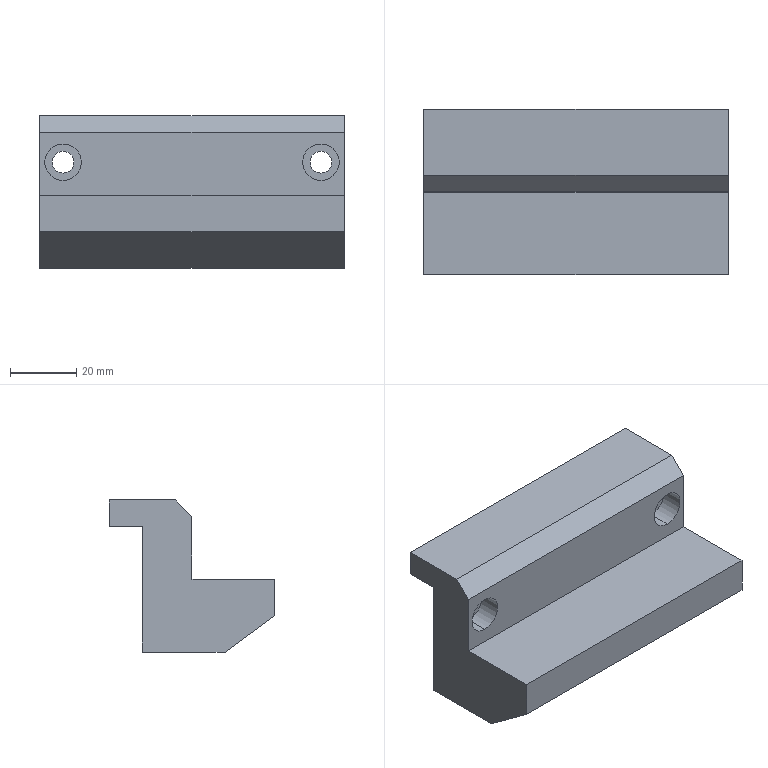Component | SolidWorks | RetractableStop-LongSide-1_AlignmentStop-0510-1 | 1 solid | 22 faces | box 92 x 50 x 46 mm | volume 110846 mm3 | plane 14 | cylinder 8 | commonest cylinder face diameters 11 x4 6.6 x4
build123d program:
from build123d import *

# Parameters (mm, degrees)
SKETCH1_W                                            = 92
SKETCH1_H                                            = 15
BOSS_EXTRUDE1_DEPTH                                  = 46
HOLE_SIZE_ACCORDING_TO_HEX_SOCKET_HEAD_C_D           = 6.6
HOLE_SIZE_ACCORDING_TO_HEX_SOCKET_HEAD_C_CBORE_D     = 11
HOLE_SIZE_ACCORDING_TO_HEX_SOCKET_HEAD_C_CBORE_DEPTH = 6.8
SKETCH11_W                                           = 92
SKETCH11_H                                           = 22
BOSS_EXTRUDE2_DEPTH                                  = 25
SKETCH12_W                                           = 92
SKETCH12_H                                           = 8
BOSS_EXTRUDE3_DEPTH                                  = 10
CUT_EXTRUDE1_DEPTH                                   = 106.854
CHAMFER1_SIZE                                        = 5


with BuildPart() as part:
    # Sketch1 → Boss-Extrude1 (new body)
    with BuildSketch(Plane.XY):
        with Locations((46, -7.5)):
            Rectangle(SKETCH1_W, SKETCH1_H)
    extrude(amount=BOSS_EXTRUDE1_DEPTH)

    # Hole Size according to Hex Socket Head C (through all)
    with Locations(Plane(origin=(0, 0, 0), x_dir=(1, 0, 0), z_dir=(0, 1, 0))):
        with Locations((7, -14), (85, -14)):
            CounterBoreHole(HOLE_SIZE_ACCORDING_TO_HEX_SOCKET_HEAD_C_D / 2, HOLE_SIZE_ACCORDING_TO_HEX_SOCKET_HEAD_C_CBORE_D / 2, HOLE_SIZE_ACCORDING_TO_HEX_SOCKET_HEAD_C_CBORE_DEPTH)

    # Sketch11 → Boss-Extrude2 (add)
    with BuildSketch(Plane(origin=(0, 0, 0), x_dir=(1, 0, 0), z_dir=(0, 1, 0))):
        with Locations((46, -35)):
            Rectangle(SKETCH11_W, SKETCH11_H)
    extrude(amount=BOSS_EXTRUDE2_DEPTH)

    # Sketch12 → Boss-Extrude3 (add)
    with BuildSketch(Plane.XZ.offset(15)):
        with Locations((46, 4)):
            Rectangle(SKETCH12_W, SKETCH12_H)
    extrude(amount=BOSS_EXTRUDE3_DEPTH)

    # Sketch13 → Cut-Extrude1 (cut, through all)
    with BuildSketch(Plane.ZY):
        Polygon((35, 25), (46, 10), (46, 25), align=None)
    extrude(amount=-CUT_EXTRUDE1_DEPTH, mode=Mode.SUBTRACT)

    # Chamfer1
    chamfer1_edges = [part.edges().sort_by_distance(p)[0] for p in [
        (46, 0, 0),
    ]]
    chamfer(chamfer1_edges, length=CHAMFER1_SIZE)


solid = part.part

# Placed as in the assembly
solid = solid.moved(Location((-1378.013, -21.764, 3640.5), (180, 0, 0)))
STEP:
#1=CARTESIAN_POINT('',(-53.977,-0.5891,142.992));
#2=VERTEX_POINT('',#1);
#3=CARTESIAN_POINT('',(-53.977,-0.5891,142.559));
#4=VERTEX_POINT('',#3);
#5=CARTESIAN_POINT('',(-53.977,-0.5891,142.776));
#6=DIRECTION('',(0.,-1.,0.));
#7=DIRECTION('',(0.,-0.,-1.));
#8=AXIS2_PLACEMENT_3D('',#5,#6,#7);
#9=CIRCLE('',#8,0.2165);
#10=EDGE_CURVE('',#2,#4,#9,.T.);
#11=ORIENTED_EDGE('',*,*,#10,.F.);
#12=CARTESIAN_POINT('',(-53.977,-0.8568,142.992));
#13=VERTEX_POINT('',#12);
#14=CARTESIAN_POINT('',(-53.977,-0.8568,142.992));
#15=DIRECTION('',(0.,-1.,0.));
#16=VECTOR('',#15,39.37);
#17=LINE('',#14,#16);
#18=EDGE_CURVE('',#2,#13,#17,.T.);
#19=ORIENTED_EDGE('',*,*,#18,.T.);
#20=CARTESIAN_POINT('',(-53.977,-0.8568,142.559));
#21=VERTEX_POINT('',#20);
#22=CARTESIAN_POINT('',(-53.977,-0.8568,142.776));
#23=DIRECTION('',(0.,-1.,0.));
#24=DIRECTION('',(0.,0.,-1.));
#25=AXIS2_PLACEMENT_3D('',#22,#23,#24);
#26=CIRCLE('',#25,0.2165);
#27=EDGE_CURVE('',#13,#21,#26,.T.);
#28=ORIENTED_EDGE('',*,*,#27,.T.);
#29=CARTESIAN_POINT('',(-53.977,-0.8568,142.559));
#30=DIRECTION('',(0.,-1.,0.));
#31=VECTOR('',#30,39.37);
#32=LINE('',#29,#31);
#33=EDGE_CURVE('',#4,#21,#32,.T.);
#34=ORIENTED_EDGE('',*,*,#33,.F.);
#35=EDGE_LOOP('',(#11,#19,#28,#34));
#36=FACE_OUTER_BOUND('',#35,.T.);
#37=CARTESIAN_POINT('',(-53.977,-0.8568,142.776));
#38=DIRECTION('',(0.,-1.,0.));
#39=DIRECTION('',(0.,0.,-1.));
#40=AXIS2_PLACEMENT_3D('',#37,#38,#39);
#41=CYLINDRICAL_SURFACE('',#40,0.2165);
#42=ADVANCED_FACE('',(#36),#41,.F.);
#43=CARTESIAN_POINT('',(-53.977,-0.2663,142.906));
#44=VERTEX_POINT('',#43);
#45=CARTESIAN_POINT('',(-53.977,-0.2663,142.646));
#46=VERTEX_POINT('',#45);
#47=CARTESIAN_POINT('',(-53.977,-0.2663,142.776));
#48=DIRECTION('',(0.,-1.,0.));
#49=DIRECTION('',(0.,-0.,-1.));
#50=AXIS2_PLACEMENT_3D('',#47,#48,#49);
#51=CIRCLE('',#50,0.1299);
#52=EDGE_CURVE('',#44,#46,#51,.T.);
#53=ORIENTED_EDGE('',*,*,#52,.F.);
#54=CARTESIAN_POINT('',(-53.977,-0.5891,142.906));
#55=VERTEX_POINT('',#54);
#56=CARTESIAN_POINT('',(-53.977,-0.8568,142.906));
#57=DIRECTION('',(0.,-1.,0.));
#58=VECTOR('',#57,39.37);
#59=LINE('',#56,#58);
#60=EDGE_CURVE('',#44,#55,#59,.T.);
#61=ORIENTED_EDGE('',*,*,#60,.T.);
#62=CARTESIAN_POINT('',(-53.977,-0.5891,142.646));
#63=VERTEX_POINT('',#62);
#64=CARTESIAN_POINT('',(-53.977,-0.5891,142.776));
#65=DIRECTION('',(0.,-1.,0.));
#66=DIRECTION('',(0.,-0.,-1.));
#67=AXIS2_PLACEMENT_3D('',#64,#65,#66);
#68=CIRCLE('',#67,0.1299);
#69=EDGE_CURVE('',#55,#63,#68,.T.);
#70=ORIENTED_EDGE('',*,*,#69,.T.);
#71=CARTESIAN_POINT('',(-53.977,-0.8568,142.646));
#72=DIRECTION('',(0.,-1.,0.));
#73=VECTOR('',#72,39.37);
#74=LINE('',#71,#73);
#75=EDGE_CURVE('',#46,#63,#74,.T.);
#76=ORIENTED_EDGE('',*,*,#75,.F.);
#77=EDGE_LOOP('',(#53,#61,#70,#76));
#78=FACE_OUTER_BOUND('',#77,.T.);
#79=CARTESIAN_POINT('',(-53.977,-0.8568,142.776));
#80=DIRECTION('',(0.,-1.,0.));
#81=DIRECTION('',(0.,0.,-1.));
#82=AXIS2_PLACEMENT_3D('',#79,#80,#81);
#83=CYLINDRICAL_SURFACE('',#82,0.1299);
#84=ADVANCED_FACE('',(#78),#83,.F.);
#85=CARTESIAN_POINT('',(-50.906,-0.5891,142.992));
#86=VERTEX_POINT('',#85);
#87=CARTESIAN_POINT('',(-50.906,-0.5891,142.559));
#88=VERTEX_POINT('',#87);
#89=CARTESIAN_POINT('',(-50.906,-0.5891,142.776));
#90=DIRECTION('',(0.,-1.,0.));
#91=DIRECTION('',(0.,-0.,-1.));
#92=AXIS2_PLACEMENT_3D('',#89,#90,#91);
#93=CIRCLE('',#92,0.2165);
#94=EDGE_CURVE('',#86,#88,#93,.T.);
#95=ORIENTED_EDGE('',*,*,#94,.F.);
#96=CARTESIAN_POINT('',(-50.906,-0.8568,142.992));
#97=VERTEX_POINT('',#96);
#98=CARTESIAN_POINT('',(-50.906,-0.8568,142.992));
#99=DIRECTION('',(0.,-1.,0.));
#100=VECTOR('',#99,39.37);
#101=LINE('',#98,#100);
#102=EDGE_CURVE('',#86,#97,#101,.T.);
#103=ORIENTED_EDGE('',*,*,#102,.T.);
#104=CARTESIAN_POINT('',(-50.906,-0.8568,142.559));
#105=VERTEX_POINT('',#104);
#106=CARTESIAN_POINT('',(-50.906,-0.8568,142.776));
#107=DIRECTION('',(0.,-1.,0.));
#108=DIRECTION('',(0.,0.,-1.));
#109=AXIS2_PLACEMENT_3D('',#106,#107,#108);
#110=CIRCLE('',#109,0.2165);
#111=EDGE_CURVE('',#97,#105,#110,.T.);
#112=ORIENTED_EDGE('',*,*,#111,.T.);
#113=CARTESIAN_POINT('',(-50.906,-0.8568,142.559));
#114=DIRECTION('',(0.,-1.,0.));
#115=VECTOR('',#114,39.37);
#116=LINE('',#113,#115);
#117=EDGE_CURVE('',#88,#105,#116,.T.);
#118=ORIENTED_EDGE('',*,*,#117,.F.);
#119=EDGE_LOOP('',(#95,#103,#112,#118));
#120=FACE_OUTER_BOUND('',#119,.T.);
#121=CARTESIAN_POINT('',(-50.906,-0.8568,142.776));
#122=DIRECTION('',(0.,-1.,0.));
#123=DIRECTION('',(0.,0.,-1.));
#124=AXIS2_PLACEMENT_3D('',#121,#122,#123);
#125=CYLINDRICAL_SURFACE('',#124,0.2165);
#126=ADVANCED_FACE('',(#120),#125,.F.);
#127=CARTESIAN_POINT('',(-50.906,-0.2663,142.906));
#128=VERTEX_POINT('',#127);
#129=CARTESIAN_POINT('',(-50.906,-0.2663,142.646));
#130=VERTEX_POINT('',#129);
#131=CARTESIAN_POINT('',(-50.906,-0.2663,142.776));
#132=DIRECTION('',(0.,-1.,0.));
#133=DIRECTION('',(0.,-0.,-1.));
#134=AXIS2_PLACEMENT_3D('',#131,#132,#133);
#135=CIRCLE('',#134,0.1299);
#136=EDGE_CURVE('',#128,#130,#135,.T.);
#137=ORIENTED_EDGE('',*,*,#136,.F.);
#138=CARTESIAN_POINT('',(-50.906,-0.5891,142.906));
#139=VERTEX_POINT('',#138);
#140=CARTESIAN_POINT('',(-50.906,-0.8568,142.906));
#141=DIRECTION('',(0.,-1.,0.));
#142=VECTOR('',#141,39.37);
#143=LINE('',#140,#142);
#144=EDGE_CURVE('',#128,#139,#143,.T.);
#145=ORIENTED_EDGE('',*,*,#144,.T.);
#146=CARTESIAN_POINT('',(-50.906,-0.5891,142.646));
#147=VERTEX_POINT('',#146);
#148=CARTESIAN_POINT('',(-50.906,-0.5891,142.776));
#149=DIRECTION('',(0.,-1.,0.));
#150=DIRECTION('',(0.,-0.,-1.));
#151=AXIS2_PLACEMENT_3D('',#148,#149,#150);
#152=CIRCLE('',#151,0.1299);
#153=EDGE_CURVE('',#139,#147,#152,.T.);
#154=ORIENTED_EDGE('',*,*,#153,.T.);
#155=CARTESIAN_POINT('',(-50.906,-0.8568,142.646));
#156=DIRECTION('',(0.,-1.,0.));
#157=VECTOR('',#156,39.37);
#158=LINE('',#155,#157);
#159=EDGE_CURVE('',#130,#147,#158,.T.);
#160=ORIENTED_EDGE('',*,*,#159,.F.);
#161=EDGE_LOOP('',(#137,#145,#154,#160));
#162=FACE_OUTER_BOUND('',#161,.T.);
#163=CARTESIAN_POINT('',(-50.906,-0.8568,142.776));
#164=DIRECTION('',(0.,-1.,0.));
#165=DIRECTION('',(0.,0.,-1.));
#166=AXIS2_PLACEMENT_3D('',#163,#164,#165);
#167=CYLINDRICAL_SURFACE('',#166,0.1299);
#168=ADVANCED_FACE('',(#162),#167,.F.);
#169=CARTESIAN_POINT('',(-50.906,-0.2663,142.776));
#170=DIRECTION('',(0.,-1.,0.));
#171=DIRECTION('',(0.,-0.,-1.));
#172=AXIS2_PLACEMENT_3D('',#169,#170,#171);
#173=CIRCLE('',#172,0.1299);
#174=EDGE_CURVE('',#130,#128,#173,.T.);
#175=ORIENTED_EDGE('',*,*,#174,.T.);
#176=ORIENTED_EDGE('',*,*,#136,.T.);
#177=EDGE_LOOP('',(#175,#176));
#178=FACE_BOUND('',#177,.T.);
#179=CARTESIAN_POINT('',(-53.977,-0.2663,142.776));
#180=DIRECTION('',(0.,-1.,0.));
#181=DIRECTION('',(0.,-0.,-1.));
#182=AXIS2_PLACEMENT_3D('',#179,#180,#181);
#183=CIRCLE('',#182,0.1299);
#184=EDGE_CURVE('',#46,#44,#183,.T.);
#185=ORIENTED_EDGE('',*,*,#184,.T.);
#186=ORIENTED_EDGE('',*,*,#52,.T.);
#187=EDGE_LOOP('',(#185,#186));
#188=FACE_BOUND('',#187,.T.);
#189=CARTESIAN_POINT('',(-50.63,-0.2663,143.012));
#190=VERTEX_POINT('',#189);
#191=CARTESIAN_POINT('',(-54.252,-0.2663,143.012));
#192=VERTEX_POINT('',#191);
#193=CARTESIAN_POINT('',(-54.252,-0.2663,143.012));
#194=DIRECTION('',(-1.,-0.,0.));
#195=VECTOR('',#194,39.37);
#196=LINE('',#193,#195);
#197=EDGE_CURVE('',#190,#192,#196,.T.);
#198=ORIENTED_EDGE('',*,*,#197,.F.);
#199=CARTESIAN_POINT('',(-50.63,-0.2663,141.516));
#200=VERTEX_POINT('',#199);
#201=CARTESIAN_POINT('',(-50.63,-0.2663,141.516));
#202=DIRECTION('',(0.,0.,1.));
#203=VECTOR('',#202,39.37);
#204=LINE('',#201,#203);
#205=EDGE_CURVE('',#200,#190,#204,.T.);
#206=ORIENTED_EDGE('',*,*,#205,.F.);
#207=CARTESIAN_POINT('',(-54.252,-0.2663,141.516));
#208=VERTEX_POINT('',#207);
#209=CARTESIAN_POINT('',(-54.252,-0.2663,141.516));
#210=DIRECTION('',(1.,0.,-0.));
#211=VECTOR('',#210,39.37);
#212=LINE('',#209,#211);
#213=EDGE_CURVE('',#208,#200,#212,.T.);
#214=ORIENTED_EDGE('',*,*,#213,.F.);
#215=CARTESIAN_POINT('',(-54.252,-0.2663,141.516));
#216=DIRECTION('',(0.,0.,1.));
#217=VECTOR('',#216,39.37);
#218=LINE('',#215,#217);
#219=EDGE_CURVE('',#208,#192,#218,.T.);
#220=ORIENTED_EDGE('',*,*,#219,.T.);
#221=EDGE_LOOP('',(#198,#206,#214,#220));
#222=FACE_OUTER_BOUND('',#221,.T.);
#223=CARTESIAN_POINT('',(-54.252,-0.2663,141.516));
#224=DIRECTION('',(0.,-1.,0.));
#225=DIRECTION('',(-1.,-0.,0.));
#226=AXIS2_PLACEMENT_3D('',#223,#224,#225);
#227=PLANE('',#226);
#228=ADVANCED_FACE('',(#178,#188,#222),#227,.F.);
#229=CARTESIAN_POINT('',(-50.906,-0.8568,142.776));
#230=DIRECTION('',(0.,-1.,0.));
#231=DIRECTION('',(0.,0.,-1.));
#232=AXIS2_PLACEMENT_3D('',#229,#230,#231);
#233=CIRCLE('',#232,0.2165);
#234=EDGE_CURVE('',#105,#97,#233,.T.);
#235=ORIENTED_EDGE('',*,*,#234,.F.);
#236=ORIENTED_EDGE('',*,*,#111,.F.);
#237=EDGE_LOOP('',(#235,#236));
#238=FACE_BOUND('',#237,.T.);
#239=CARTESIAN_POINT('',(-53.977,-0.8568,142.776));
#240=DIRECTION('',(0.,-1.,0.));
#241=DIRECTION('',(0.,0.,-1.));
#242=AXIS2_PLACEMENT_3D('',#239,#240,#241);
#243=CIRCLE('',#242,0.2165);
#244=EDGE_CURVE('',#21,#13,#243,.T.);
#245=ORIENTED_EDGE('',*,*,#244,.F.);
#246=ORIENTED_EDGE('',*,*,#27,.F.);
#247=EDGE_LOOP('',(#245,#246));
#248=FACE_BOUND('',#247,.T.);
#249=CARTESIAN_POINT('',(-50.63,-0.8568,142.382));
#250=VERTEX_POINT('',#249);
#251=CARTESIAN_POINT('',(-50.63,-0.8568,143.13));
#252=VERTEX_POINT('',#251);
#253=CARTESIAN_POINT('',(-50.63,-0.8568,141.516));
#254=DIRECTION('',(0.,0.,1.));
#255=VECTOR('',#254,39.37);
#256=LINE('',#253,#255);
#257=EDGE_CURVE('',#250,#252,#256,.T.);
#258=ORIENTED_EDGE('',*,*,#257,.T.);
#259=CARTESIAN_POINT('',(-54.252,-0.8568,143.13));
#260=VERTEX_POINT('',#259);
#261=CARTESIAN_POINT('',(-50.63,-0.8568,143.13));
#262=DIRECTION('',(-1.,0.,0.));
#263=VECTOR('',#262,39.37);
#264=LINE('',#261,#263);
#265=EDGE_CURVE('',#252,#260,#264,.T.);
#266=ORIENTED_EDGE('',*,*,#265,.T.);
#267=CARTESIAN_POINT('',(-54.252,-0.8568,142.382));
#268=VERTEX_POINT('',#267);
#269=CARTESIAN_POINT('',(-54.252,-0.8568,141.516));
#270=DIRECTION('',(0.,0.,1.));
#271=VECTOR('',#270,39.37);
#272=LINE('',#269,#271);
#273=EDGE_CURVE('',#268,#260,#272,.T.);
#274=ORIENTED_EDGE('',*,*,#273,.F.);
#275=CARTESIAN_POINT('',(-54.252,-0.8568,142.382));
#276=DIRECTION('',(-1.,0.,0.));
#277=VECTOR('',#276,39.37);
#278=LINE('',#275,#277);
#279=EDGE_CURVE('',#250,#268,#278,.T.);
#280=ORIENTED_EDGE('',*,*,#279,.F.);
#281=EDGE_LOOP('',(#258,#266,#274,#280));
#282=FACE_OUTER_BOUND('',#281,.T.);
#283=CARTESIAN_POINT('',(-50.63,-0.8568,141.516));
#284=DIRECTION('',(0.,1.,-0.));
#285=DIRECTION('',(1.,-0.,-0.));
#286=AXIS2_PLACEMENT_3D('',#283,#284,#285);
#287=PLANE('',#286);
#288=ADVANCED_FACE('',(#238,#248,#282),#287,.F.);
#289=CARTESIAN_POINT('',(-50.63,0.1274,143.327));
#290=VERTEX_POINT('',#289);
#291=CARTESIAN_POINT('',(-50.63,-0.66,143.327));
#292=VERTEX_POINT('',#291);
#293=CARTESIAN_POINT('',(-50.63,-0.2663,143.327));
#294=DIRECTION('',(0.,-1.,0.));
#295=VECTOR('',#294,39.37);
#296=LINE('',#293,#295);
#297=EDGE_CURVE('',#290,#292,#296,.T.);
#298=ORIENTED_EDGE('',*,*,#297,.T.);
#299=CARTESIAN_POINT('',(-50.63,-0.8568,143.13));
#300=DIRECTION('',(-0.,-0.7071,-0.7071));
#301=VECTOR('',#300,39.37);
#302=LINE('',#299,#301);
#303=EDGE_CURVE('',#292,#252,#302,.T.);
#304=ORIENTED_EDGE('',*,*,#303,.T.);
#305=ORIENTED_EDGE('',*,*,#257,.F.);
#306=CARTESIAN_POINT('',(-50.63,-1.841,142.382));
#307=VERTEX_POINT('',#306);
#308=CARTESIAN_POINT('',(-50.63,-1.841,142.382));
#309=DIRECTION('',(0.,1.,-0.));
#310=VECTOR('',#309,39.37);
#311=LINE('',#308,#310);
#312=EDGE_CURVE('',#307,#250,#311,.T.);
#313=ORIENTED_EDGE('',*,*,#312,.F.);
#314=CARTESIAN_POINT('',(-50.63,-1.841,141.949));
#315=VERTEX_POINT('',#314);
#316=CARTESIAN_POINT('',(-50.63,-1.841,141.516));
#317=DIRECTION('',(0.,0.,1.));
#318=VECTOR('',#317,39.37);
#319=LINE('',#316,#318);
#320=EDGE_CURVE('',#315,#307,#319,.T.);
#321=ORIENTED_EDGE('',*,*,#320,.F.);
#322=CARTESIAN_POINT('',(-50.63,-1.251,141.516));
#323=VERTEX_POINT('',#322);
#324=CARTESIAN_POINT('',(-50.63,-0.6105,141.046));
#325=DIRECTION('',(-0.,0.8064,-0.5914));
#326=VECTOR('',#325,39.37);
#327=LINE('',#324,#326);
#328=EDGE_CURVE('',#315,#323,#327,.T.);
#329=ORIENTED_EDGE('',*,*,#328,.T.);
#330=CARTESIAN_POINT('',(-50.63,-0.2663,141.516));
#331=DIRECTION('',(0.,-1.,0.));
#332=VECTOR('',#331,39.37);
#333=LINE('',#330,#332);
#334=EDGE_CURVE('',#200,#323,#333,.T.);
#335=ORIENTED_EDGE('',*,*,#334,.F.);
#336=ORIENTED_EDGE('',*,*,#205,.T.);
#337=CARTESIAN_POINT('',(-50.63,0.1274,143.012));
#338=VERTEX_POINT('',#337);
#339=CARTESIAN_POINT('',(-50.63,0.1274,143.012));
#340=DIRECTION('',(0.,-1.,0.));
#341=VECTOR('',#340,39.37);
#342=LINE('',#339,#341);
#343=EDGE_CURVE('',#338,#190,#342,.T.);
#344=ORIENTED_EDGE('',*,*,#343,.F.);
#345=CARTESIAN_POINT('',(-50.63,0.1274,143.327));
#346=DIRECTION('',(-0.,-0.,-1.));
#347=VECTOR('',#346,39.37);
#348=LINE('',#345,#347);
#349=EDGE_CURVE('',#290,#338,#348,.T.);
#350=ORIENTED_EDGE('',*,*,#349,.F.);
#351=EDGE_LOOP('',(#298,#304,#305,#313,#321,#329,#335,#336,#344,#350));
#352=FACE_OUTER_BOUND('',#351,.T.);
#353=CARTESIAN_POINT('',(-50.63,-0.2663,141.516));
#354=DIRECTION('',(-1.,-0.,0.));
#355=DIRECTION('',(-0.,-0.,-1.));
#356=AXIS2_PLACEMENT_3D('',#353,#354,#355);
#357=PLANE('',#356);
#358=ADVANCED_FACE('',(#352),#357,.F.);
#359=ORIENTED_EDGE('',*,*,#273,.T.);
#360=CARTESIAN_POINT('',(-54.252,-0.66,143.327));
#361=VERTEX_POINT('',#360);
#362=CARTESIAN_POINT('',(-54.252,-0.8568,143.13));
#363=DIRECTION('',(0.,0.7071,0.7071));
#364=VECTOR('',#363,39.37);
#365=LINE('',#362,#364);
#366=EDGE_CURVE('',#260,#361,#365,.T.);
#367=ORIENTED_EDGE('',*,*,#366,.T.);
#368=CARTESIAN_POINT('',(-54.252,0.1274,143.327));
#369=VERTEX_POINT('',#368);
#370=CARTESIAN_POINT('',(-54.252,-0.8568,143.327));
#371=DIRECTION('',(-0.,1.,-0.));
#372=VECTOR('',#371,39.37);
#373=LINE('',#370,#372);
#374=EDGE_CURVE('',#361,#369,#373,.T.);
#375=ORIENTED_EDGE('',*,*,#374,.T.);
#376=CARTESIAN_POINT('',(-54.252,0.1274,143.012));
#377=VERTEX_POINT('',#376);
#378=CARTESIAN_POINT('',(-54.252,0.1274,143.327));
#379=DIRECTION('',(0.,0.,1.));
#380=VECTOR('',#379,39.37);
#381=LINE('',#378,#380);
#382=EDGE_CURVE('',#377,#369,#381,.T.);
#383=ORIENTED_EDGE('',*,*,#382,.F.);
#384=CARTESIAN_POINT('',(-54.252,0.1274,143.012));
#385=DIRECTION('',(0.,-1.,0.));
#386=VECTOR('',#385,39.37);
#387=LINE('',#384,#386);
#388=EDGE_CURVE('',#377,#192,#387,.T.);
#389=ORIENTED_EDGE('',*,*,#388,.T.);
#390=ORIENTED_EDGE('',*,*,#219,.F.);
#391=CARTESIAN_POINT('',(-54.252,-1.251,141.516));
#392=VERTEX_POINT('',#391);
#393=CARTESIAN_POINT('',(-54.252,-0.8568,141.516));
#394=DIRECTION('',(-0.,1.,-0.));
#395=VECTOR('',#394,39.37);
#396=LINE('',#393,#395);
#397=EDGE_CURVE('',#392,#208,#396,.T.);
#398=ORIENTED_EDGE('',*,*,#397,.F.);
#399=CARTESIAN_POINT('',(-54.252,-1.841,141.949));
#400=VERTEX_POINT('',#399);
#401=CARTESIAN_POINT('',(-54.252,-1.841,141.949));
#402=DIRECTION('',(-0.,0.8064,-0.5914));
#403=VECTOR('',#402,39.37);
#404=LINE('',#401,#403);
#405=EDGE_CURVE('',#400,#392,#404,.T.);
#406=ORIENTED_EDGE('',*,*,#405,.F.);
#407=CARTESIAN_POINT('',(-54.252,-1.841,142.382));
#408=VERTEX_POINT('',#407);
#409=CARTESIAN_POINT('',(-54.252,-1.841,141.516));
#410=DIRECTION('',(-0.,-0.,-1.));
#411=VECTOR('',#410,39.37);
#412=LINE('',#409,#411);
#413=EDGE_CURVE('',#408,#400,#412,.T.);
#414=ORIENTED_EDGE('',*,*,#413,.F.);
#415=CARTESIAN_POINT('',(-54.252,-1.841,142.382));
#416=DIRECTION('',(0.,1.,-0.));
#417=VECTOR('',#416,39.37);
#418=LINE('',#415,#417);
#419=EDGE_CURVE('',#408,#268,#418,.T.);
#420=ORIENTED_EDGE('',*,*,#419,.T.);
#421=EDGE_LOOP('',(#359,#367,#375,#383,#389,#390,#398,#406,#414,#420));
#422=FACE_OUTER_BOUND('',#421,.T.);
#423=CARTESIAN_POINT('',(-54.252,-0.8568,141.516));
#424=DIRECTION('',(1.,0.,-0.));
#425=DIRECTION('',(0.,0.,1.));
#426=AXIS2_PLACEMENT_3D('',#423,#424,#425);
#427=PLANE('',#426);
#428=ADVANCED_FACE('',(#422),#427,.F.);
#429=CARTESIAN_POINT('',(-50.63,-1.251,141.516));
#430=DIRECTION('',(-1.,-0.,0.));
#431=VECTOR('',#430,39.37);
#432=LINE('',#429,#431);
#433=EDGE_CURVE('',#323,#392,#432,.T.);
#434=ORIENTED_EDGE('',*,*,#433,.T.);
#435=ORIENTED_EDGE('',*,*,#397,.T.);
#436=ORIENTED_EDGE('',*,*,#213,.T.);
#437=ORIENTED_EDGE('',*,*,#334,.T.);
#438=EDGE_LOOP('',(#434,#435,#436,#437));
#439=FACE_OUTER_BOUND('',#438,.T.);
#440=CARTESIAN_POINT('',(-54.252,-0.8568,141.516));
#441=DIRECTION('',(-0.,-0.,-1.));
#442=DIRECTION('',(1.,0.,-0.));
#443=AXIS2_PLACEMENT_3D('',#440,#441,#442);
#444=PLANE('',#443);
#445=ADVANCED_FACE('',(#439),#444,.T.);
#446=ORIENTED_EDGE('',*,*,#374,.F.);
#447=CARTESIAN_POINT('',(-54.252,-0.66,143.327));
#448=DIRECTION('',(1.,-0.,-0.));
#449=VECTOR('',#448,39.37);
#450=LINE('',#447,#449);
#451=EDGE_CURVE('',#361,#292,#450,.T.);
#452=ORIENTED_EDGE('',*,*,#451,.T.);
#453=ORIENTED_EDGE('',*,*,#297,.F.);
#454=CARTESIAN_POINT('',(-54.252,0.1274,143.327));
#455=DIRECTION('',(1.,0.,-0.));
#456=VECTOR('',#455,39.37);
#457=LINE('',#454,#456);
#458=EDGE_CURVE('',#369,#290,#457,.T.);
#459=ORIENTED_EDGE('',*,*,#458,.F.);
#460=EDGE_LOOP('',(#446,#452,#453,#459));
#461=FACE_OUTER_BOUND('',#460,.T.);
#462=CARTESIAN_POINT('',(-54.252,-0.8568,143.327));
#463=DIRECTION('',(-0.,-0.,-1.));
#464=DIRECTION('',(1.,0.,-0.));
#465=AXIS2_PLACEMENT_3D('',#462,#463,#464);
#466=PLANE('',#465);
#467=ADVANCED_FACE('',(#461),#466,.F.);
#468=ORIENTED_EDGE('',*,*,#144,.F.);
#469=ORIENTED_EDGE('',*,*,#174,.F.);
#470=ORIENTED_EDGE('',*,*,#159,.T.);
#471=CARTESIAN_POINT('',(-50.906,-0.5891,142.776));
#472=DIRECTION('',(0.,-1.,0.));
#473=DIRECTION('',(0.,-0.,-1.));
#474=AXIS2_PLACEMENT_3D('',#471,#472,#473);
#475=CIRCLE('',#474,0.1299);
#476=EDGE_CURVE('',#147,#139,#475,.T.);
#477=ORIENTED_EDGE('',*,*,#476,.T.);
#478=EDGE_LOOP('',(#468,#469,#470,#477));
#479=FACE_OUTER_BOUND('',#478,.T.);
#480=CARTESIAN_POINT('',(-50.906,-0.8568,142.776));
#481=DIRECTION('',(0.,-1.,0.));
#482=DIRECTION('',(0.,0.,-1.));
#483=AXIS2_PLACEMENT_3D('',#480,#481,#482);
#484=CYLINDRICAL_SURFACE('',#483,0.1299);
#485=ADVANCED_FACE('',(#479),#484,.F.);
#486=ORIENTED_EDGE('',*,*,#476,.F.);
#487=ORIENTED_EDGE('',*,*,#153,.F.);
#488=EDGE_LOOP('',(#486,#487));
#489=FACE_BOUND('',#488,.T.);
#490=CARTESIAN_POINT('',(-50.906,-0.5891,142.776));
#491=DIRECTION('',(0.,-1.,0.));
#492=DIRECTION('',(0.,-0.,-1.));
#493=AXIS2_PLACEMENT_3D('',#490,#491,#492);
#494=CIRCLE('',#493,0.2165);
#495=EDGE_CURVE('',#88,#86,#494,.T.);
#496=ORIENTED_EDGE('',*,*,#495,.T.);
#497=ORIENTED_EDGE('',*,*,#94,.T.);
#498=EDGE_LOOP('',(#496,#497));
#499=FACE_OUTER_BOUND('',#498,.T.);
#500=CARTESIAN_POINT('',(-50.776,-0.5891,142.776));
#501=DIRECTION('',(-0.,1.,-0.));
#502=DIRECTION('',(0.,0.,1.));
#503=AXIS2_PLACEMENT_3D('',#500,#501,#502);
#504=PLANE('',#503);
#505=ADVANCED_FACE('',(#489,#499),#504,.F.);
#506=ORIENTED_EDGE('',*,*,#102,.F.);
#507=ORIENTED_EDGE('',*,*,#495,.F.);
#508=ORIENTED_EDGE('',*,*,#117,.T.);
#509=ORIENTED_EDGE('',*,*,#234,.T.);
#510=EDGE_LOOP('',(#506,#507,#508,#509));
#511=FACE_OUTER_BOUND('',#510,.T.);
#512=CARTESIAN_POINT('',(-50.906,-0.8568,142.776));
#513=DIRECTION('',(0.,-1.,0.));
#514=DIRECTION('',(0.,0.,-1.));
#515=AXIS2_PLACEMENT_3D('',#512,#513,#514);
#516=CYLINDRICAL_SURFACE('',#515,0.2165);
#517=ADVANCED_FACE('',(#511),#516,.F.);
#518=ORIENTED_EDGE('',*,*,#60,.F.);
#519=ORIENTED_EDGE('',*,*,#184,.F.);
#520=ORIENTED_EDGE('',*,*,#75,.T.);
#521=CARTESIAN_POINT('',(-53.977,-0.5891,142.776));
#522=DIRECTION('',(0.,-1.,0.));
#523=DIRECTION('',(0.,-0.,-1.));
#524=AXIS2_PLACEMENT_3D('',#521,#522,#523);
#525=CIRCLE('',#524,0.1299);
#526=EDGE_CURVE('',#63,#55,#525,.T.);
#527=ORIENTED_EDGE('',*,*,#526,.T.);
#528=EDGE_LOOP('',(#518,#519,#520,#527));
#529=FACE_OUTER_BOUND('',#528,.T.);
#530=CARTESIAN_POINT('',(-53.977,-0.8568,142.776));
#531=DIRECTION('',(0.,-1.,0.));
#532=DIRECTION('',(0.,0.,-1.));
#533=AXIS2_PLACEMENT_3D('',#530,#531,#532);
#534=CYLINDRICAL_SURFACE('',#533,0.1299);
#535=ADVANCED_FACE('',(#529),#534,.F.);
#536=ORIENTED_EDGE('',*,*,#526,.F.);
#537=ORIENTED_EDGE('',*,*,#69,.F.);
#538=EDGE_LOOP('',(#536,#537));
#539=FACE_BOUND('',#538,.T.);
#540=CARTESIAN_POINT('',(-53.977,-0.5891,142.776));
#541=DIRECTION('',(0.,-1.,0.));
#542=DIRECTION('',(0.,-0.,-1.));
#543=AXIS2_PLACEMENT_3D('',#540,#541,#542);
#544=CIRCLE('',#543,0.2165);
#545=EDGE_CURVE('',#4,#2,#544,.T.);
#546=ORIENTED_EDGE('',*,*,#545,.T.);
#547=ORIENTED_EDGE('',*,*,#10,.T.);
#548=EDGE_LOOP('',(#546,#547));
#549=FACE_OUTER_BOUND('',#548,.T.);
#550=CARTESIAN_POINT('',(-53.847,-0.5891,142.776));
#551=DIRECTION('',(-0.,1.,-0.));
#552=DIRECTION('',(0.,0.,1.));
#553=AXIS2_PLACEMENT_3D('',#550,#551,#552);
#554=PLANE('',#553);
#555=ADVANCED_FACE('',(#539,#549),#554,.F.);
#556=ORIENTED_EDGE('',*,*,#18,.F.);
#557=ORIENTED_EDGE('',*,*,#545,.F.);
#558=ORIENTED_EDGE('',*,*,#33,.T.);
#559=ORIENTED_EDGE('',*,*,#244,.T.);
#560=EDGE_LOOP('',(#556,#557,#558,#559));
#561=FACE_OUTER_BOUND('',#560,.T.);
#562=CARTESIAN_POINT('',(-53.977,-0.8568,142.776));
#563=DIRECTION('',(0.,-1.,0.));
#564=DIRECTION('',(0.,0.,-1.));
#565=AXIS2_PLACEMENT_3D('',#562,#563,#564);
#566=CYLINDRICAL_SURFACE('',#565,0.2165);
#567=ADVANCED_FACE('',(#561),#566,.F.);
#568=ORIENTED_EDGE('',*,*,#279,.T.);
#569=ORIENTED_EDGE('',*,*,#419,.F.);
#570=CARTESIAN_POINT('',(-54.252,-1.841,142.382));
#571=DIRECTION('',(-1.,0.,0.));
#572=VECTOR('',#571,39.37);
#573=LINE('',#570,#572);
#574=EDGE_CURVE('',#307,#408,#573,.T.);
#575=ORIENTED_EDGE('',*,*,#574,.F.);
#576=ORIENTED_EDGE('',*,*,#312,.T.);
#577=EDGE_LOOP('',(#568,#569,#575,#576));
#578=FACE_OUTER_BOUND('',#577,.T.);
#579=CARTESIAN_POINT('',(-54.252,-1.841,142.382));
#580=DIRECTION('',(-0.,-0.,-1.));
#581=DIRECTION('',(1.,0.,-0.));
#582=AXIS2_PLACEMENT_3D('',#579,#580,#581);
#583=PLANE('',#582);
#584=ADVANCED_FACE('',(#578),#583,.F.);
#585=ORIENTED_EDGE('',*,*,#413,.T.);
#586=CARTESIAN_POINT('',(-54.252,-1.841,141.949));
#587=DIRECTION('',(1.,-0.,-0.));
#588=VECTOR('',#587,39.37);
#589=LINE('',#586,#588);
#590=EDGE_CURVE('',#400,#315,#589,.T.);
#591=ORIENTED_EDGE('',*,*,#590,.T.);
#592=ORIENTED_EDGE('',*,*,#320,.T.);
#593=ORIENTED_EDGE('',*,*,#574,.T.);
#594=EDGE_LOOP('',(#585,#591,#592,#593));
#595=FACE_OUTER_BOUND('',#594,.T.);
#596=CARTESIAN_POINT('',(-54.252,-1.841,143.327));
#597=DIRECTION('',(0.,1.,-0.));
#598=DIRECTION('',(1.,-0.,-0.));
#599=AXIS2_PLACEMENT_3D('',#596,#597,#598);
#600=PLANE('',#599);
#601=ADVANCED_FACE('',(#595),#600,.F.);
#602=ORIENTED_EDGE('',*,*,#197,.T.);
#603=ORIENTED_EDGE('',*,*,#388,.F.);
#604=CARTESIAN_POINT('',(-54.252,0.1274,143.012));
#605=DIRECTION('',(-1.,-0.,0.));
#606=VECTOR('',#605,39.37);
#607=LINE('',#604,#606);
#608=EDGE_CURVE('',#338,#377,#607,.T.);
#609=ORIENTED_EDGE('',*,*,#608,.F.);
#610=ORIENTED_EDGE('',*,*,#343,.T.);
#611=EDGE_LOOP('',(#602,#603,#609,#610));
#612=FACE_OUTER_BOUND('',#611,.T.);
#613=CARTESIAN_POINT('',(-54.252,0.1274,143.012));
#614=DIRECTION('',(0.,0.,1.));
#615=DIRECTION('',(-1.,-0.,0.));
#616=AXIS2_PLACEMENT_3D('',#613,#614,#615);
#617=PLANE('',#616);
#618=ADVANCED_FACE('',(#612),#617,.F.);
#619=ORIENTED_EDGE('',*,*,#382,.T.);
#620=ORIENTED_EDGE('',*,*,#458,.T.);
#621=ORIENTED_EDGE('',*,*,#349,.T.);
#622=ORIENTED_EDGE('',*,*,#608,.T.);
#623=EDGE_LOOP('',(#619,#620,#621,#622));
#624=FACE_OUTER_BOUND('',#623,.T.);
#625=CARTESIAN_POINT('',(-54.252,0.1274,143.327));
#626=DIRECTION('',(0.,-1.,0.));
#627=DIRECTION('',(-1.,-0.,0.));
#628=AXIS2_PLACEMENT_3D('',#625,#626,#627);
#629=PLANE('',#628);
#630=ADVANCED_FACE('',(#624),#629,.F.);
#631=ORIENTED_EDGE('',*,*,#590,.F.);
#632=ORIENTED_EDGE('',*,*,#405,.T.);
#633=ORIENTED_EDGE('',*,*,#433,.F.);
#634=ORIENTED_EDGE('',*,*,#328,.F.);
#635=EDGE_LOOP('',(#631,#632,#633,#634));
#636=FACE_OUTER_BOUND('',#635,.T.);
#637=CARTESIAN_POINT('',(-50.63,-1.841,141.949));
#638=DIRECTION('',(0.,0.5914,0.8064));
#639=DIRECTION('',(0.,-0.8064,0.5914));
#640=AXIS2_PLACEMENT_3D('',#637,#638,#639);
#641=PLANE('',#640);
#642=ADVANCED_FACE('',(#636),#641,.F.);
#643=ORIENTED_EDGE('',*,*,#303,.F.);
#644=ORIENTED_EDGE('',*,*,#451,.F.);
#645=ORIENTED_EDGE('',*,*,#366,.F.);
#646=ORIENTED_EDGE('',*,*,#265,.F.);
#647=EDGE_LOOP('',(#643,#644,#645,#646));
#648=FACE_OUTER_BOUND('',#647,.T.);
#649=CARTESIAN_POINT('',(-50.63,-0.8568,143.13));
#650=DIRECTION('',(-0.,0.7071,-0.7071));
#651=DIRECTION('',(-1.,0.,0.));
#652=AXIS2_PLACEMENT_3D('',#649,#650,#651);
#653=PLANE('',#652);
#654=ADVANCED_FACE('',(#648),#653,.F.);
#655=CLOSED_SHELL('',(#42,#84,#126,#168,#228,#288,#358,#428,#445,#467,#485,#505,#517,#535,#555,#567,#584,#601,#618,#630,#642,#654));
#656=MANIFOLD_SOLID_BREP('',#655);
#657=CARTESIAN_POINT('',(0.,0.,0.));
#658=DIRECTION('',(0.,0.,1.));
#659=DIRECTION('',(1.,0.,0.));
#660=AXIS2_PLACEMENT_3D('',#657,#658,#659);
#661=(LENGTH_UNIT()NAMED_UNIT(*)SI_UNIT($,.METRE.));
#662=LENGTH_MEASURE_WITH_UNIT(LENGTH_MEASURE(0.0254),#661);
#663=DIMENSIONAL_EXPONENTS(1.,0.,0.,0.,0.,0.,0.);
#664=(CONVERSION_BASED_UNIT('',#662)LENGTH_UNIT()NAMED_UNIT(#663));
#665=UNCERTAINTY_MEASURE_WITH_UNIT(LENGTH_MEASURE(0.00001),#664,'','');
#666=(NAMED_UNIT(*)PLANE_ANGLE_UNIT()SI_UNIT($,.RADIAN.));
#667=(NAMED_UNIT(*)SI_UNIT($,.STERADIAN.)SOLID_ANGLE_UNIT());
#668=(GEOMETRIC_REPRESENTATION_CONTEXT(3)GLOBAL_UNCERTAINTY_ASSIGNED_CONTEXT((#665))GLOBAL_UNIT_ASSIGNED_CONTEXT((#664,#666,#667))REPRESENTATION_CONTEXT('',''));
#669=ADVANCED_BREP_SHAPE_REPRESENTATION('',(#656,#660),#668);
#670=COLOUR_RGB('',0.7922,0.8196,0.9333);
#671=FILL_AREA_STYLE_COLOUR('',#670);
#672=FILL_AREA_STYLE('',(#671));
#673=SURFACE_STYLE_FILL_AREA(#672);
#674=SURFACE_SIDE_STYLE('',(#673));
#675=SURFACE_STYLE_USAGE(.BOTH.,#674);
#676=PRESENTATION_STYLE_ASSIGNMENT((#675));
#677=STYLED_ITEM('',(#676),#656);
#678=(LENGTH_UNIT()NAMED_UNIT(*)SI_UNIT($,.METRE.));
#679=LENGTH_MEASURE_WITH_UNIT(LENGTH_MEASURE(0.0254),#678);
#680=DIMENSIONAL_EXPONENTS(1.,0.,0.,0.,0.,0.,0.);
#681=(CONVERSION_BASED_UNIT('',#679)LENGTH_UNIT()NAMED_UNIT(#680));
#682=UNCERTAINTY_MEASURE_WITH_UNIT(LENGTH_MEASURE(0.00001),#681,'','');
#683=(NAMED_UNIT(*)PLANE_ANGLE_UNIT()SI_UNIT($,.RADIAN.));
#684=(NAMED_UNIT(*)SI_UNIT($,.STERADIAN.)SOLID_ANGLE_UNIT());
#685=(GEOMETRIC_REPRESENTATION_CONTEXT(3)GLOBAL_UNCERTAINTY_ASSIGNED_CONTEXT((#682))GLOBAL_UNIT_ASSIGNED_CONTEXT((#681,#683,#684))REPRESENTATION_CONTEXT('',''));
#686=MECHANICAL_DESIGN_GEOMETRIC_PRESENTATION_REPRESENTATION('',(#677),#685);
#687=PRESENTATION_LAYER_ASSIGNMENT('','',(#677));